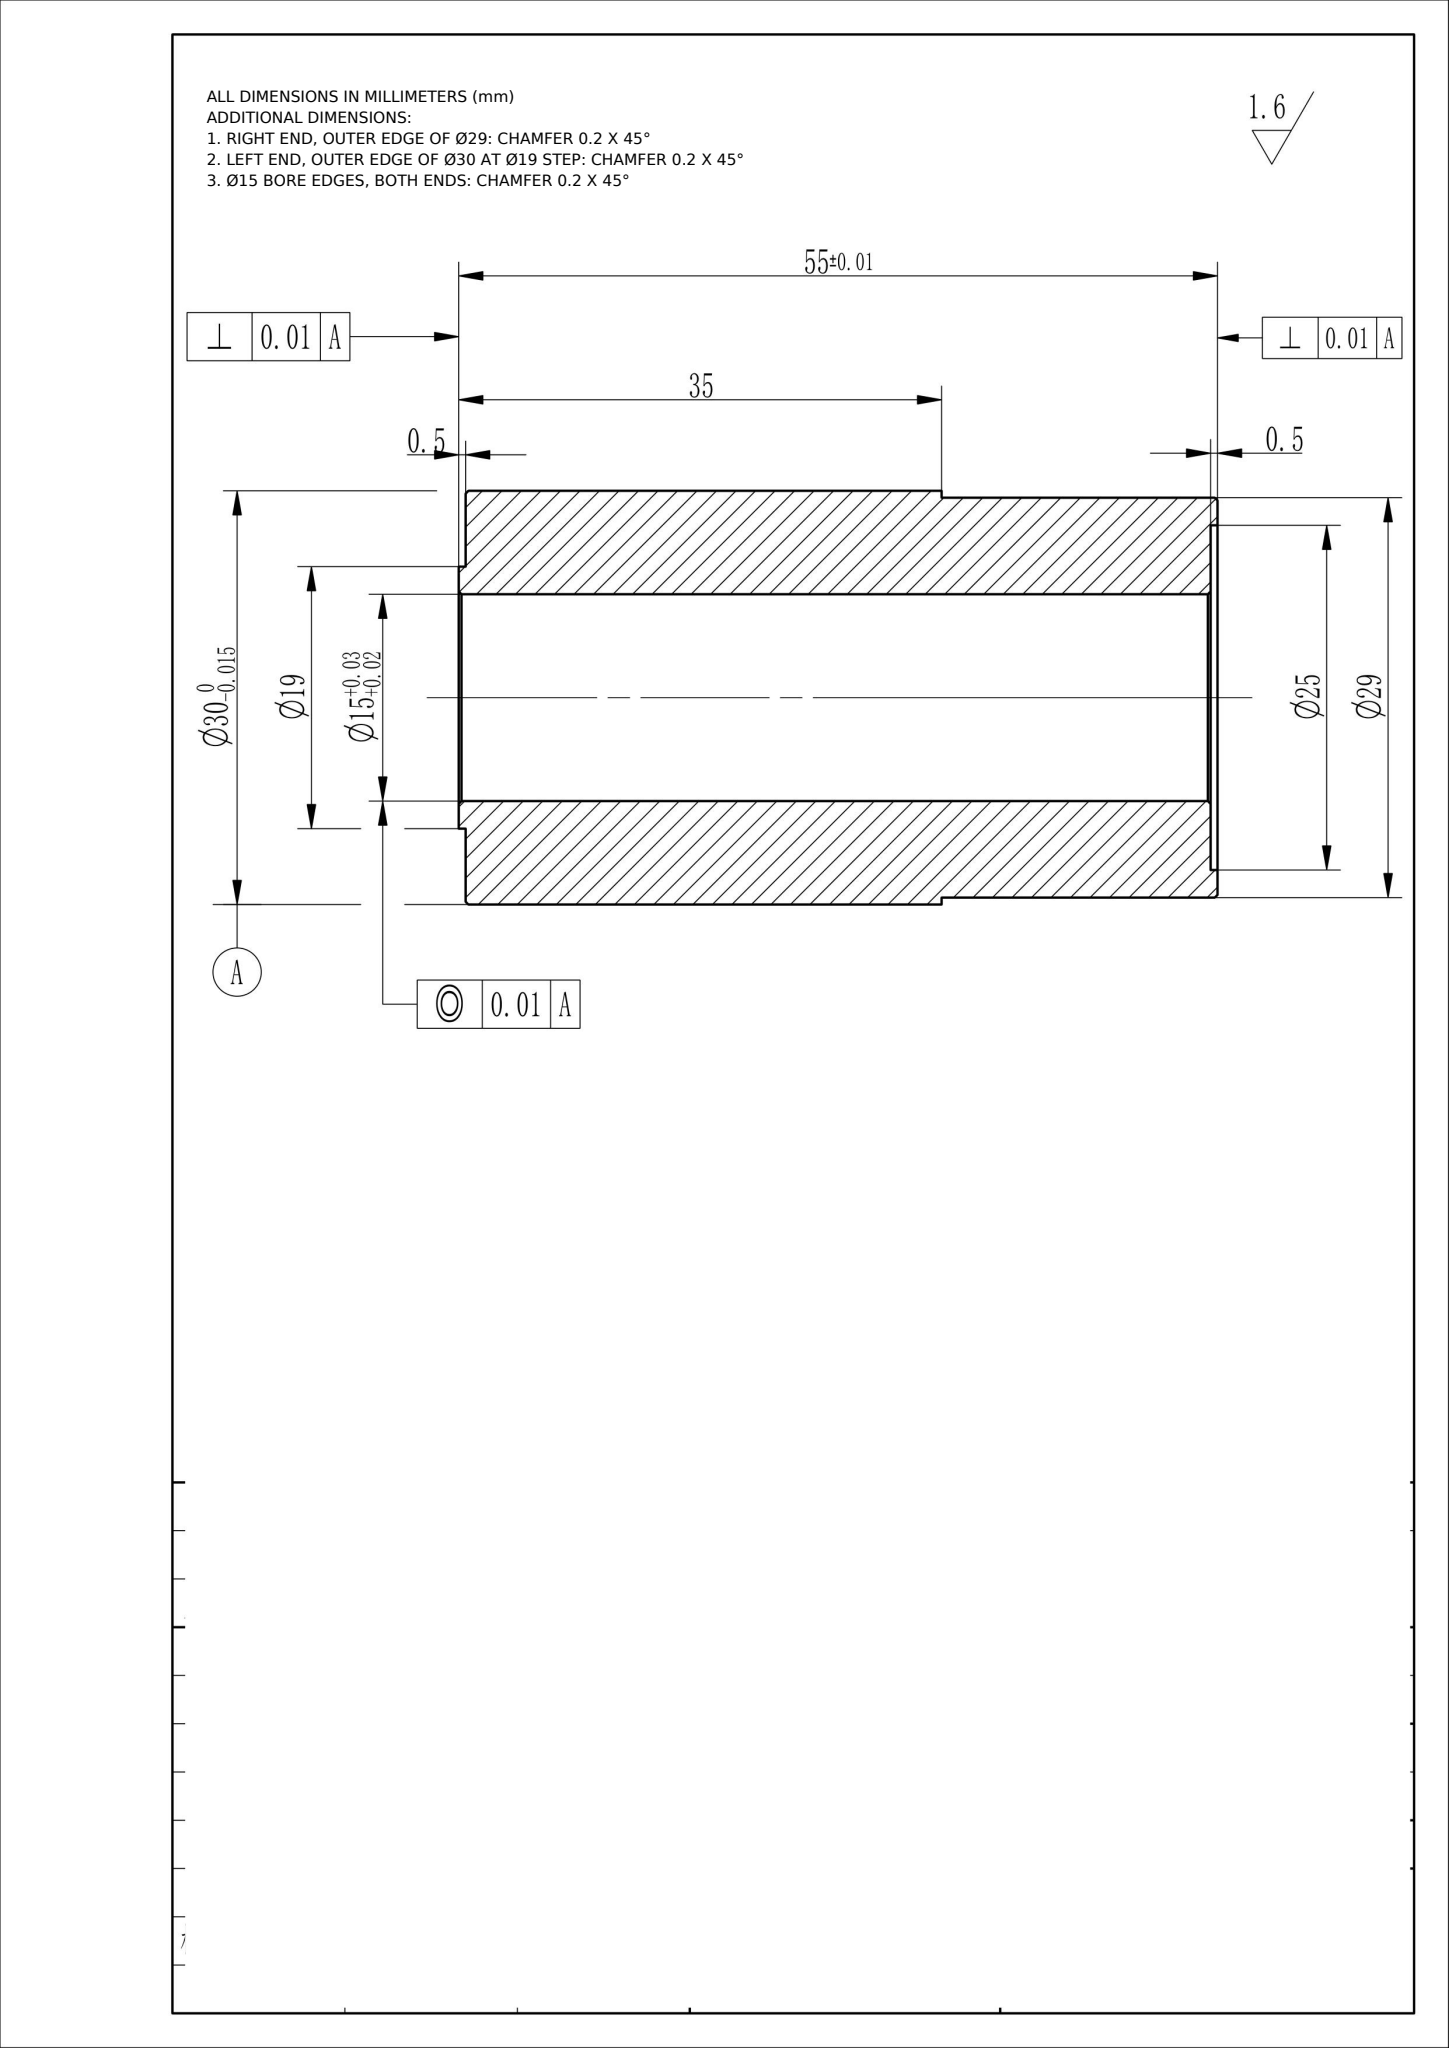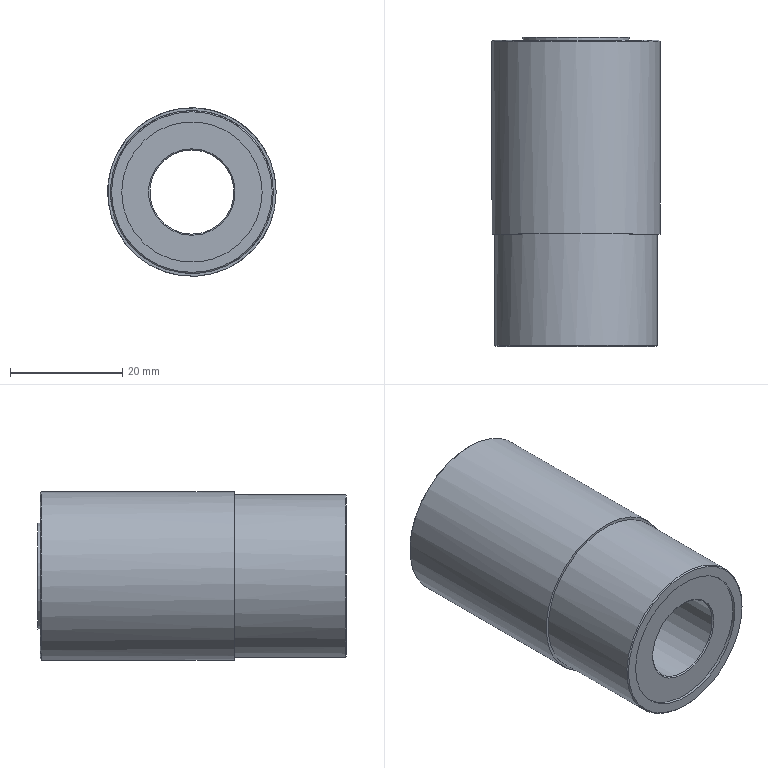Part | NX | mm | 1 solid | 14 faces | box 30 x 55 x 30 mm | volume 27857 mm3 | cylinder 5 | plane 5 | cone 4 | commonest cylinder face diameters 30 x1 15 x1 19 x1 25 x1 29 x1
STEP:
#1=CARTESIAN_POINT('',(0.,0.,0.));
#2=DIRECTION('',(0.,0.,1.));
#3=DIRECTION('',(1.,0.,0.));
#4=AXIS2_PLACEMENT_3D('',#1,#2,#3);
#5=(LENGTH_UNIT()NAMED_UNIT(*)SI_UNIT(.MILLI.,.METRE.));
#6=UNCERTAINTY_MEASURE_WITH_UNIT(LENGTH_MEASURE(0.00002),#5,'','');
#7=(NAMED_UNIT(*)PLANE_ANGLE_UNIT()SI_UNIT($,.RADIAN.));
#8=PLANE_ANGLE_MEASURE_WITH_UNIT(PLANE_ANGLE_MEASURE(0.01745),#7);
#9=DIMENSIONAL_EXPONENTS(0.,0.,0.,0.,0.,0.,0.);
#10=(CONVERSION_BASED_UNIT('',#8)NAMED_UNIT(#9)PLANE_ANGLE_UNIT());
#11=(NAMED_UNIT(*)SI_UNIT($,.STERADIAN.)SOLID_ANGLE_UNIT());
#12=(GEOMETRIC_REPRESENTATION_CONTEXT(3)GLOBAL_UNCERTAINTY_ASSIGNED_CONTEXT((#6))GLOBAL_UNIT_ASSIGNED_CONTEXT((#5,#10,#11))REPRESENTATION_CONTEXT('',''));
#13=SHAPE_REPRESENTATION('',(#4),#12);
#14=CARTESIAN_POINT('',(0.,24.3,15.));
#15=VERTEX_POINT('',#14);
#16=CARTESIAN_POINT('',(0.,24.3,0.));
#17=DIRECTION('',(0.,-1.,0.));
#18=DIRECTION('',(0.,0.,1.));
#19=AXIS2_PLACEMENT_3D('',#16,#17,#18);
#20=CIRCLE('',#19,15.);
#21=EDGE_CURVE('',#15,#15,#20,.T.);
#22=ORIENTED_EDGE('',*,*,#21,.T.);
#23=EDGE_LOOP('',(#22));
#24=FACE_BOUND('',#23,.T.);
#25=CARTESIAN_POINT('',(15.,-10.,-0.));
#26=VERTEX_POINT('',#25);
#27=CARTESIAN_POINT('',(0.,-10.,0.));
#28=DIRECTION('',(0.,-1.,0.));
#29=DIRECTION('',(1.,0.,-0.));
#30=AXIS2_PLACEMENT_3D('',#27,#28,#29);
#31=CIRCLE('',#30,15.);
#32=EDGE_CURVE('',#26,#26,#31,.T.);
#33=ORIENTED_EDGE('',*,*,#32,.F.);
#34=EDGE_LOOP('',(#33));
#35=FACE_BOUND('',#34,.T.);
#36=CARTESIAN_POINT('',(0.,0.,0.));
#37=DIRECTION('',(0.,-1.,0.));
#38=DIRECTION('',(0.,0.,-1.));
#39=AXIS2_PLACEMENT_3D('',#36,#37,#38);
#40=CYLINDRICAL_SURFACE('',#39,15.);
#41=ADVANCED_FACE('',(#24,#35),#40,.T.);
#42=CARTESIAN_POINT('',(0.,-30.,14.3));
#43=VERTEX_POINT('',#42);
#44=CARTESIAN_POINT('',(0.,-30.,0.));
#45=DIRECTION('',(0.,-1.,0.));
#46=DIRECTION('',(0.,0.,1.));
#47=AXIS2_PLACEMENT_3D('',#44,#45,#46);
#48=CIRCLE('',#47,14.3);
#49=EDGE_CURVE('',#43,#43,#48,.T.);
#50=ORIENTED_EDGE('',*,*,#49,.T.);
#51=EDGE_LOOP('',(#50));
#52=FACE_BOUND('',#51,.T.);
#53=CARTESIAN_POINT('',(12.5,-30.,-0.));
#54=VERTEX_POINT('',#53);
#55=CARTESIAN_POINT('',(0.,-30.,0.));
#56=DIRECTION('',(0.,-1.,0.));
#57=DIRECTION('',(1.,0.,-0.));
#58=AXIS2_PLACEMENT_3D('',#55,#56,#57);
#59=CIRCLE('',#58,12.5);
#60=EDGE_CURVE('',#54,#54,#59,.T.);
#61=ORIENTED_EDGE('',*,*,#60,.F.);
#62=EDGE_LOOP('',(#61));
#63=FACE_BOUND('',#62,.T.);
#64=CARTESIAN_POINT('',(0.,-30.,15.));
#65=DIRECTION('',(0.,1.,0.));
#66=DIRECTION('',(0.,0.,1.));
#67=AXIS2_PLACEMENT_3D('',#64,#65,#66);
#68=PLANE('',#67);
#69=ADVANCED_FACE('',(#52,#63),#68,.F.);
#70=CARTESIAN_POINT('',(0.,25.,-7.7));
#71=VERTEX_POINT('',#70);
#72=CARTESIAN_POINT('',(0.,25.,0.));
#73=DIRECTION('',(0.,-1.,0.));
#74=DIRECTION('',(0.,0.,-1.));
#75=AXIS2_PLACEMENT_3D('',#72,#73,#74);
#76=CIRCLE('',#75,7.7);
#77=EDGE_CURVE('',#71,#71,#76,.T.);
#78=ORIENTED_EDGE('',*,*,#77,.T.);
#79=EDGE_LOOP('',(#78));
#80=FACE_BOUND('',#79,.T.);
#81=CARTESIAN_POINT('',(9.5,25.,0.));
#82=VERTEX_POINT('',#81);
#83=CARTESIAN_POINT('',(0.,25.,0.));
#84=DIRECTION('',(0.,1.,0.));
#85=DIRECTION('',(1.,0.,0.));
#86=AXIS2_PLACEMENT_3D('',#83,#84,#85);
#87=CIRCLE('',#86,9.5);
#88=EDGE_CURVE('',#82,#82,#87,.T.);
#89=ORIENTED_EDGE('',*,*,#88,.T.);
#90=EDGE_LOOP('',(#89));
#91=FACE_BOUND('',#90,.T.);
#92=CARTESIAN_POINT('',(0.,25.,7.5));
#93=DIRECTION('',(0.,-1.,0.));
#94=DIRECTION('',(0.,0.,-1.));
#95=AXIS2_PLACEMENT_3D('',#92,#93,#94);
#96=PLANE('',#95);
#97=ADVANCED_FACE('',(#80,#91),#96,.F.);
#98=CARTESIAN_POINT('',(0.,24.8,-7.5));
#99=VERTEX_POINT('',#98);
#100=CARTESIAN_POINT('',(0.,24.8,0.));
#101=DIRECTION('',(0.,1.,0.));
#102=DIRECTION('',(0.,0.,-1.));
#103=AXIS2_PLACEMENT_3D('',#100,#101,#102);
#104=CIRCLE('',#103,7.5);
#105=EDGE_CURVE('',#99,#99,#104,.T.);
#106=ORIENTED_EDGE('',*,*,#105,.T.);
#107=EDGE_LOOP('',(#106));
#108=FACE_BOUND('',#107,.T.);
#109=CARTESIAN_POINT('',(0.,-29.3,-7.5));
#110=VERTEX_POINT('',#109);
#111=CARTESIAN_POINT('',(0.,-29.3,0.));
#112=DIRECTION('',(0.,-1.,0.));
#113=DIRECTION('',(0.,0.,-1.));
#114=AXIS2_PLACEMENT_3D('',#111,#112,#113);
#115=CIRCLE('',#114,7.5);
#116=EDGE_CURVE('',#110,#110,#115,.T.);
#117=ORIENTED_EDGE('',*,*,#116,.T.);
#118=EDGE_LOOP('',(#117));
#119=FACE_BOUND('',#118,.T.);
#120=CARTESIAN_POINT('',(0.,0.,0.));
#121=DIRECTION('',(0.,-1.,0.));
#122=DIRECTION('',(0.,0.,-1.));
#123=AXIS2_PLACEMENT_3D('',#120,#121,#122);
#124=CYLINDRICAL_SURFACE('',#123,7.5);
#125=ADVANCED_FACE('',(#108,#119),#124,.F.);
#126=CARTESIAN_POINT('',(9.5,24.5,0.));
#127=VERTEX_POINT('',#126);
#128=CARTESIAN_POINT('',(0.,24.5,0.));
#129=DIRECTION('',(0.,-1.,0.));
#130=DIRECTION('',(1.,0.,0.));
#131=AXIS2_PLACEMENT_3D('',#128,#129,#130);
#132=CIRCLE('',#131,9.5);
#133=EDGE_CURVE('',#127,#127,#132,.T.);
#134=ORIENTED_EDGE('',*,*,#133,.F.);
#135=EDGE_LOOP('',(#134));
#136=FACE_BOUND('',#135,.T.);
#137=ORIENTED_EDGE('',*,*,#88,.F.);
#138=EDGE_LOOP('',(#137));
#139=FACE_BOUND('',#138,.T.);
#140=CARTESIAN_POINT('',(0.,24.5,0.));
#141=DIRECTION('',(0.,1.,0.));
#142=DIRECTION('',(0.,0.,1.));
#143=AXIS2_PLACEMENT_3D('',#140,#141,#142);
#144=CYLINDRICAL_SURFACE('',#143,9.5);
#145=ADVANCED_FACE('',(#136,#139),#144,.T.);
#146=CARTESIAN_POINT('',(0.,24.5,14.8));
#147=VERTEX_POINT('',#146);
#148=CARTESIAN_POINT('',(0.,24.5,0.));
#149=DIRECTION('',(0.,1.,0.));
#150=DIRECTION('',(0.,0.,1.));
#151=AXIS2_PLACEMENT_3D('',#148,#149,#150);
#152=CIRCLE('',#151,14.8);
#153=EDGE_CURVE('',#147,#147,#152,.T.);
#154=ORIENTED_EDGE('',*,*,#153,.T.);
#155=EDGE_LOOP('',(#154));
#156=FACE_BOUND('',#155,.T.);
#157=ORIENTED_EDGE('',*,*,#133,.T.);
#158=EDGE_LOOP('',(#157));
#159=FACE_BOUND('',#158,.T.);
#160=CARTESIAN_POINT('',(0.,24.5,0.));
#161=DIRECTION('',(0.,1.,0.));
#162=DIRECTION('',(0.,0.,1.));
#163=AXIS2_PLACEMENT_3D('',#160,#161,#162);
#164=PLANE('',#163);
#165=ADVANCED_FACE('',(#156,#159),#164,.T.);
#166=CARTESIAN_POINT('',(12.5,-29.5,-0.));
#167=VERTEX_POINT('',#166);
#168=CARTESIAN_POINT('',(0.,-29.5,0.));
#169=DIRECTION('',(0.,1.,0.));
#170=DIRECTION('',(1.,0.,-0.));
#171=AXIS2_PLACEMENT_3D('',#168,#169,#170);
#172=CIRCLE('',#171,12.5);
#173=EDGE_CURVE('',#167,#167,#172,.T.);
#174=ORIENTED_EDGE('',*,*,#173,.T.);
#175=EDGE_LOOP('',(#174));
#176=FACE_BOUND('',#175,.T.);
#177=ORIENTED_EDGE('',*,*,#60,.T.);
#178=EDGE_LOOP('',(#177));
#179=FACE_BOUND('',#178,.T.);
#180=CARTESIAN_POINT('',(0.,-29.5,0.));
#181=DIRECTION('',(0.,-1.,0.));
#182=DIRECTION('',(0.,0.,-1.));
#183=AXIS2_PLACEMENT_3D('',#180,#181,#182);
#184=CYLINDRICAL_SURFACE('',#183,12.5);
#185=ADVANCED_FACE('',(#176,#179),#184,.F.);
#186=CARTESIAN_POINT('',(0.,-29.5,-7.7));
#187=VERTEX_POINT('',#186);
#188=CARTESIAN_POINT('',(0.,-29.5,0.));
#189=DIRECTION('',(0.,1.,0.));
#190=DIRECTION('',(0.,0.,-1.));
#191=AXIS2_PLACEMENT_3D('',#188,#189,#190);
#192=CIRCLE('',#191,7.7);
#193=EDGE_CURVE('',#187,#187,#192,.T.);
#194=ORIENTED_EDGE('',*,*,#193,.T.);
#195=EDGE_LOOP('',(#194));
#196=FACE_BOUND('',#195,.T.);
#197=ORIENTED_EDGE('',*,*,#173,.F.);
#198=EDGE_LOOP('',(#197));
#199=FACE_BOUND('',#198,.T.);
#200=CARTESIAN_POINT('',(0.,-29.5,0.));
#201=DIRECTION('',(0.,-1.,0.));
#202=DIRECTION('',(0.,0.,-1.));
#203=AXIS2_PLACEMENT_3D('',#200,#201,#202);
#204=PLANE('',#203);
#205=ADVANCED_FACE('',(#196,#199),#204,.T.);
#206=ORIENTED_EDGE('',*,*,#105,.F.);
#207=EDGE_LOOP('',(#206));
#208=FACE_BOUND('',#207,.T.);
#209=ORIENTED_EDGE('',*,*,#77,.F.);
#210=EDGE_LOOP('',(#209));
#211=FACE_BOUND('',#210,.T.);
#212=CARTESIAN_POINT('',(0.,25.,0.));
#213=DIRECTION('',(0.,1.,0.));
#214=DIRECTION('',(0.,-0.,1.));
#215=AXIS2_PLACEMENT_3D('',#212,#213,#214);
#216=CONICAL_SURFACE('',#215,7.7,45.);
#217=ADVANCED_FACE('',(#208,#211),#216,.F.);
#218=ORIENTED_EDGE('',*,*,#21,.F.);
#219=EDGE_LOOP('',(#218));
#220=FACE_BOUND('',#219,.T.);
#221=ORIENTED_EDGE('',*,*,#153,.F.);
#222=EDGE_LOOP('',(#221));
#223=FACE_BOUND('',#222,.T.);
#224=CARTESIAN_POINT('',(0.,24.5,0.));
#225=DIRECTION('',(0.,-1.,0.));
#226=DIRECTION('',(0.,-0.,-1.));
#227=AXIS2_PLACEMENT_3D('',#224,#225,#226);
#228=CONICAL_SURFACE('',#227,14.8,45.);
#229=ADVANCED_FACE('',(#220,#223),#228,.T.);
#230=ORIENTED_EDGE('',*,*,#193,.F.);
#231=EDGE_LOOP('',(#230));
#232=FACE_BOUND('',#231,.T.);
#233=ORIENTED_EDGE('',*,*,#116,.F.);
#234=EDGE_LOOP('',(#233));
#235=FACE_BOUND('',#234,.T.);
#236=CARTESIAN_POINT('',(0.,-29.3,0.));
#237=DIRECTION('',(0.,-1.,0.));
#238=DIRECTION('',(0.,-0.,-1.));
#239=AXIS2_PLACEMENT_3D('',#236,#237,#238);
#240=CONICAL_SURFACE('',#239,7.5,45.);
#241=ADVANCED_FACE('',(#232,#235),#240,.F.);
#242=CARTESIAN_POINT('',(0.,-29.8,14.5));
#243=VERTEX_POINT('',#242);
#244=CARTESIAN_POINT('',(0.,-29.8,0.));
#245=DIRECTION('',(0.,1.,0.));
#246=DIRECTION('',(0.,0.,1.));
#247=AXIS2_PLACEMENT_3D('',#244,#245,#246);
#248=CIRCLE('',#247,14.5);
#249=EDGE_CURVE('',#243,#243,#248,.T.);
#250=ORIENTED_EDGE('',*,*,#249,.T.);
#251=EDGE_LOOP('',(#250));
#252=FACE_BOUND('',#251,.T.);
#253=CARTESIAN_POINT('',(14.5,-10.,-0.));
#254=VERTEX_POINT('',#253);
#255=CARTESIAN_POINT('',(0.,-10.,0.));
#256=DIRECTION('',(0.,1.,0.));
#257=DIRECTION('',(1.,0.,-0.));
#258=AXIS2_PLACEMENT_3D('',#255,#256,#257);
#259=CIRCLE('',#258,14.5);
#260=EDGE_CURVE('',#254,#254,#259,.T.);
#261=ORIENTED_EDGE('',*,*,#260,.F.);
#262=EDGE_LOOP('',(#261));
#263=FACE_BOUND('',#262,.T.);
#264=CARTESIAN_POINT('',(0.,-10.,0.));
#265=DIRECTION('',(0.,-1.,0.));
#266=DIRECTION('',(0.,0.,-1.));
#267=AXIS2_PLACEMENT_3D('',#264,#265,#266);
#268=CYLINDRICAL_SURFACE('',#267,14.5);
#269=ADVANCED_FACE('',(#252,#263),#268,.T.);
#270=ORIENTED_EDGE('',*,*,#32,.T.);
#271=EDGE_LOOP('',(#270));
#272=FACE_BOUND('',#271,.T.);
#273=ORIENTED_EDGE('',*,*,#260,.T.);
#274=EDGE_LOOP('',(#273));
#275=FACE_BOUND('',#274,.T.);
#276=CARTESIAN_POINT('',(0.,-10.,0.));
#277=DIRECTION('',(0.,-1.,0.));
#278=DIRECTION('',(0.,0.,-1.));
#279=AXIS2_PLACEMENT_3D('',#276,#277,#278);
#280=PLANE('',#279);
#281=ADVANCED_FACE('',(#272,#275),#280,.T.);
#282=ORIENTED_EDGE('',*,*,#249,.F.);
#283=EDGE_LOOP('',(#282));
#284=FACE_BOUND('',#283,.T.);
#285=ORIENTED_EDGE('',*,*,#49,.F.);
#286=EDGE_LOOP('',(#285));
#287=FACE_BOUND('',#286,.T.);
#288=CARTESIAN_POINT('',(0.,-30.,0.));
#289=DIRECTION('',(0.,1.,0.));
#290=DIRECTION('',(0.,-0.,1.));
#291=AXIS2_PLACEMENT_3D('',#288,#289,#290);
#292=CONICAL_SURFACE('',#291,14.3,45.);
#293=ADVANCED_FACE('',(#284,#287),#292,.T.);
#294=CLOSED_SHELL('',(#41,#69,#97,#125,#145,#165,#185,#205,#217,#229,#241,#269,#281,#293));
#295=MANIFOLD_SOLID_BREP('',#294);
#296=ADVANCED_BREP_SHAPE_REPRESENTATION('',(#295),#12);
#297=SHAPE_REPRESENTATION_RELATIONSHIP('','',#13,#296);
#298=PRESENTATION_LAYER_ASSIGNMENT('','',(#295));
#299=COLOUR_RGB('',1.,0.6,0.);
#300=FILL_AREA_STYLE_COLOUR('',#299);
#301=FILL_AREA_STYLE('',(#300));
#302=SURFACE_STYLE_FILL_AREA(#301);
#303=SURFACE_SIDE_STYLE('',(#302));
#304=SURFACE_STYLE_USAGE(.BOTH.,#303);
#305=PRESENTATION_STYLE_ASSIGNMENT((#304));
#306=STYLED_ITEM('',(#305),#295);
#307=MECHANICAL_DESIGN_GEOMETRIC_PRESENTATION_REPRESENTATION('',(#306),#12);